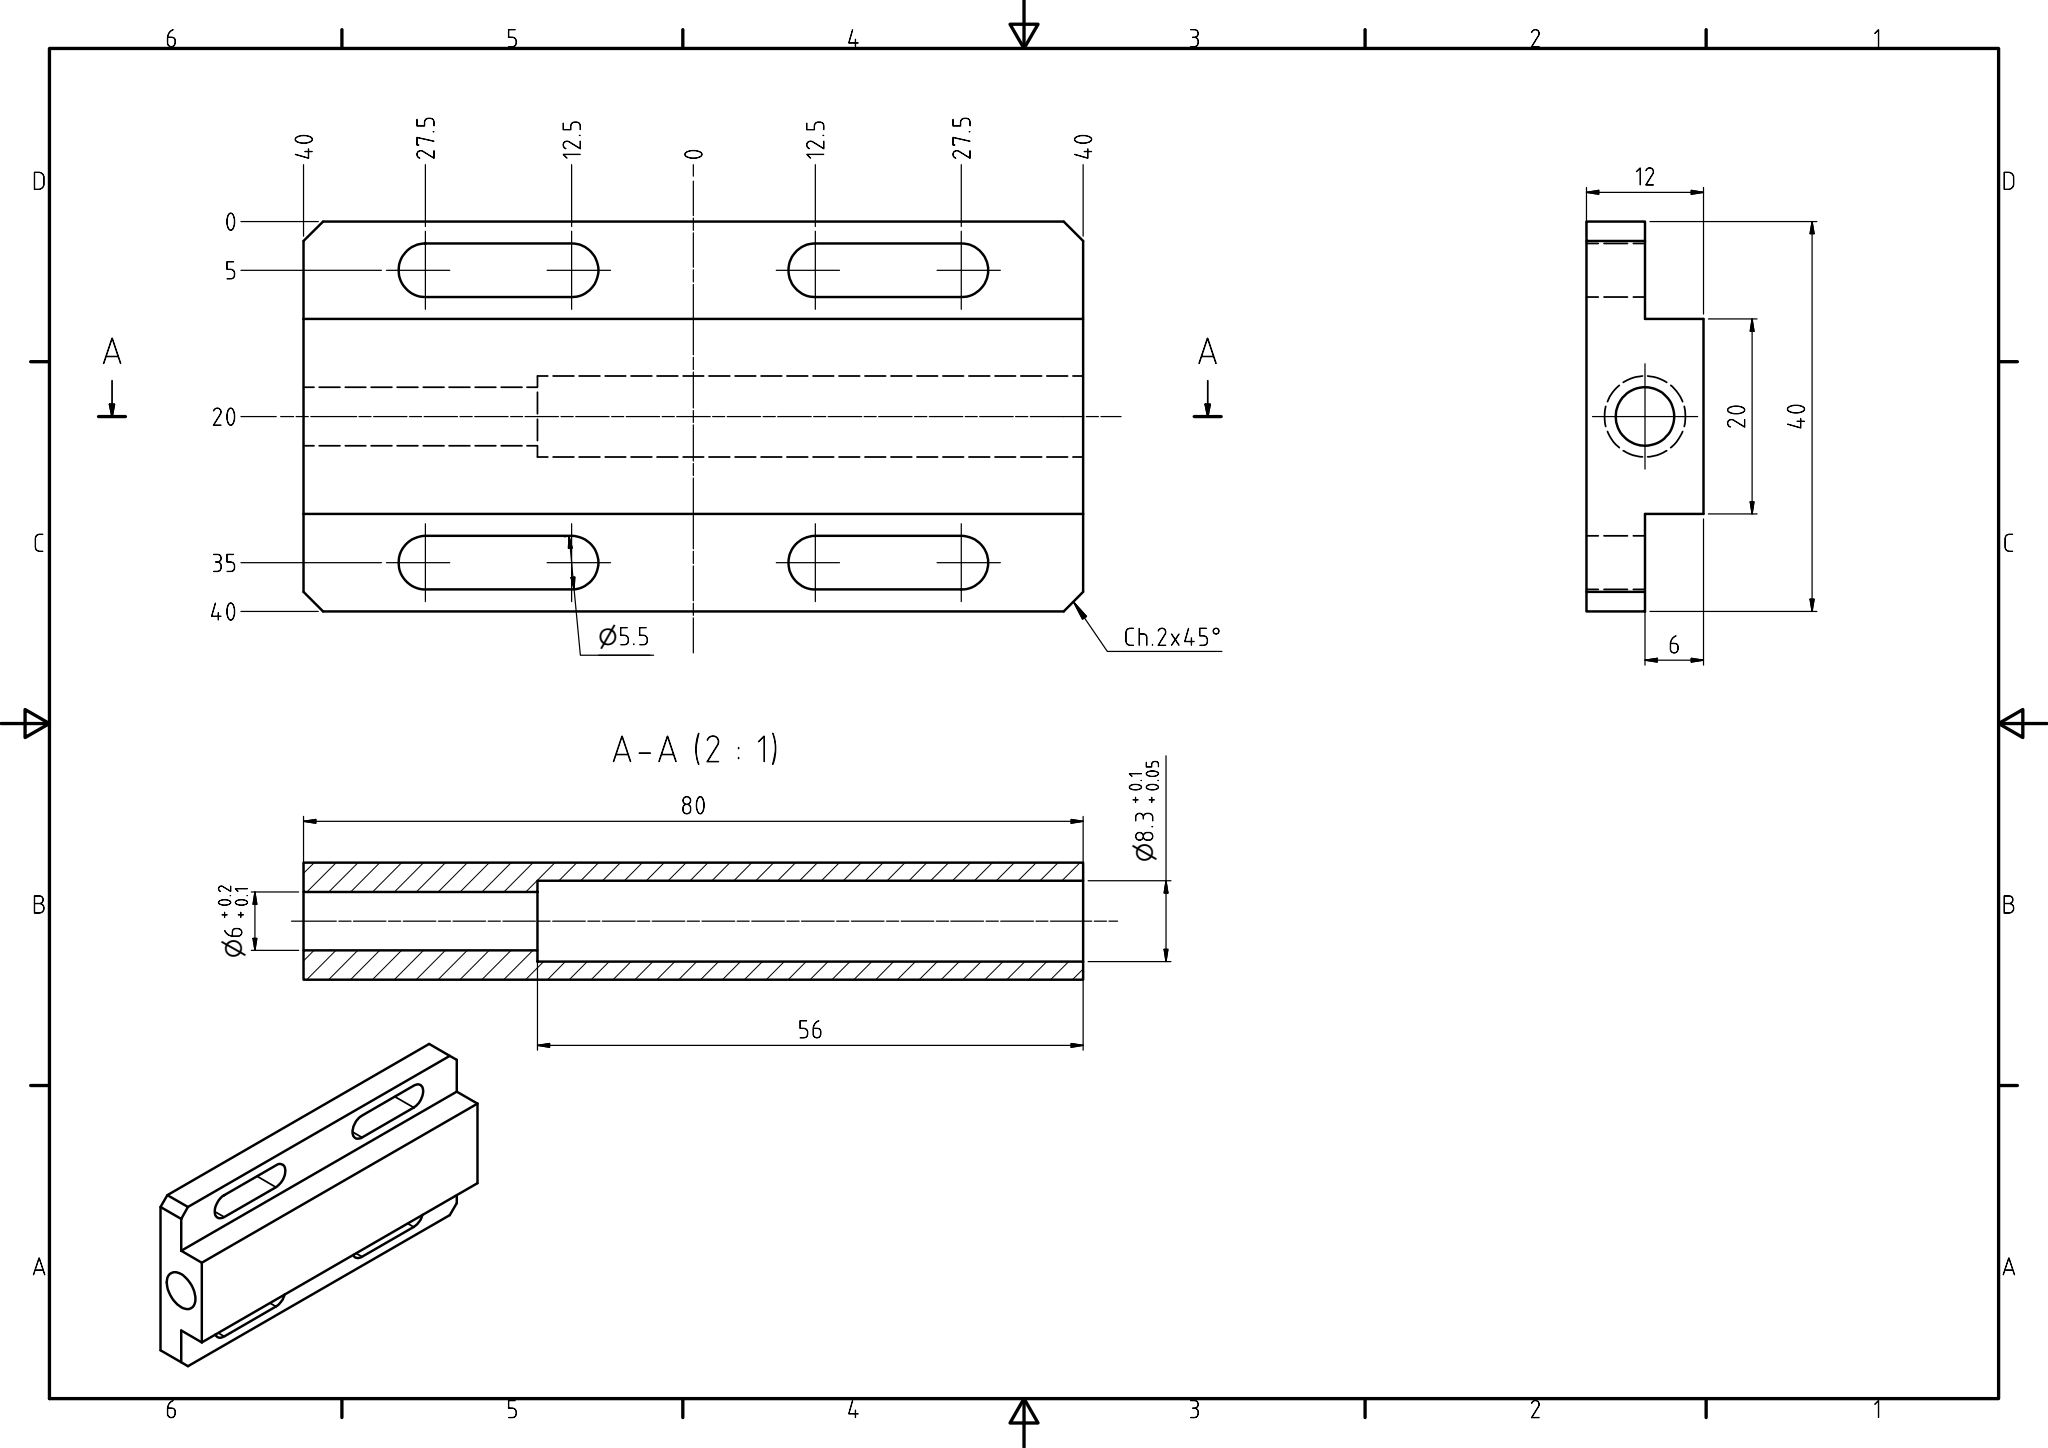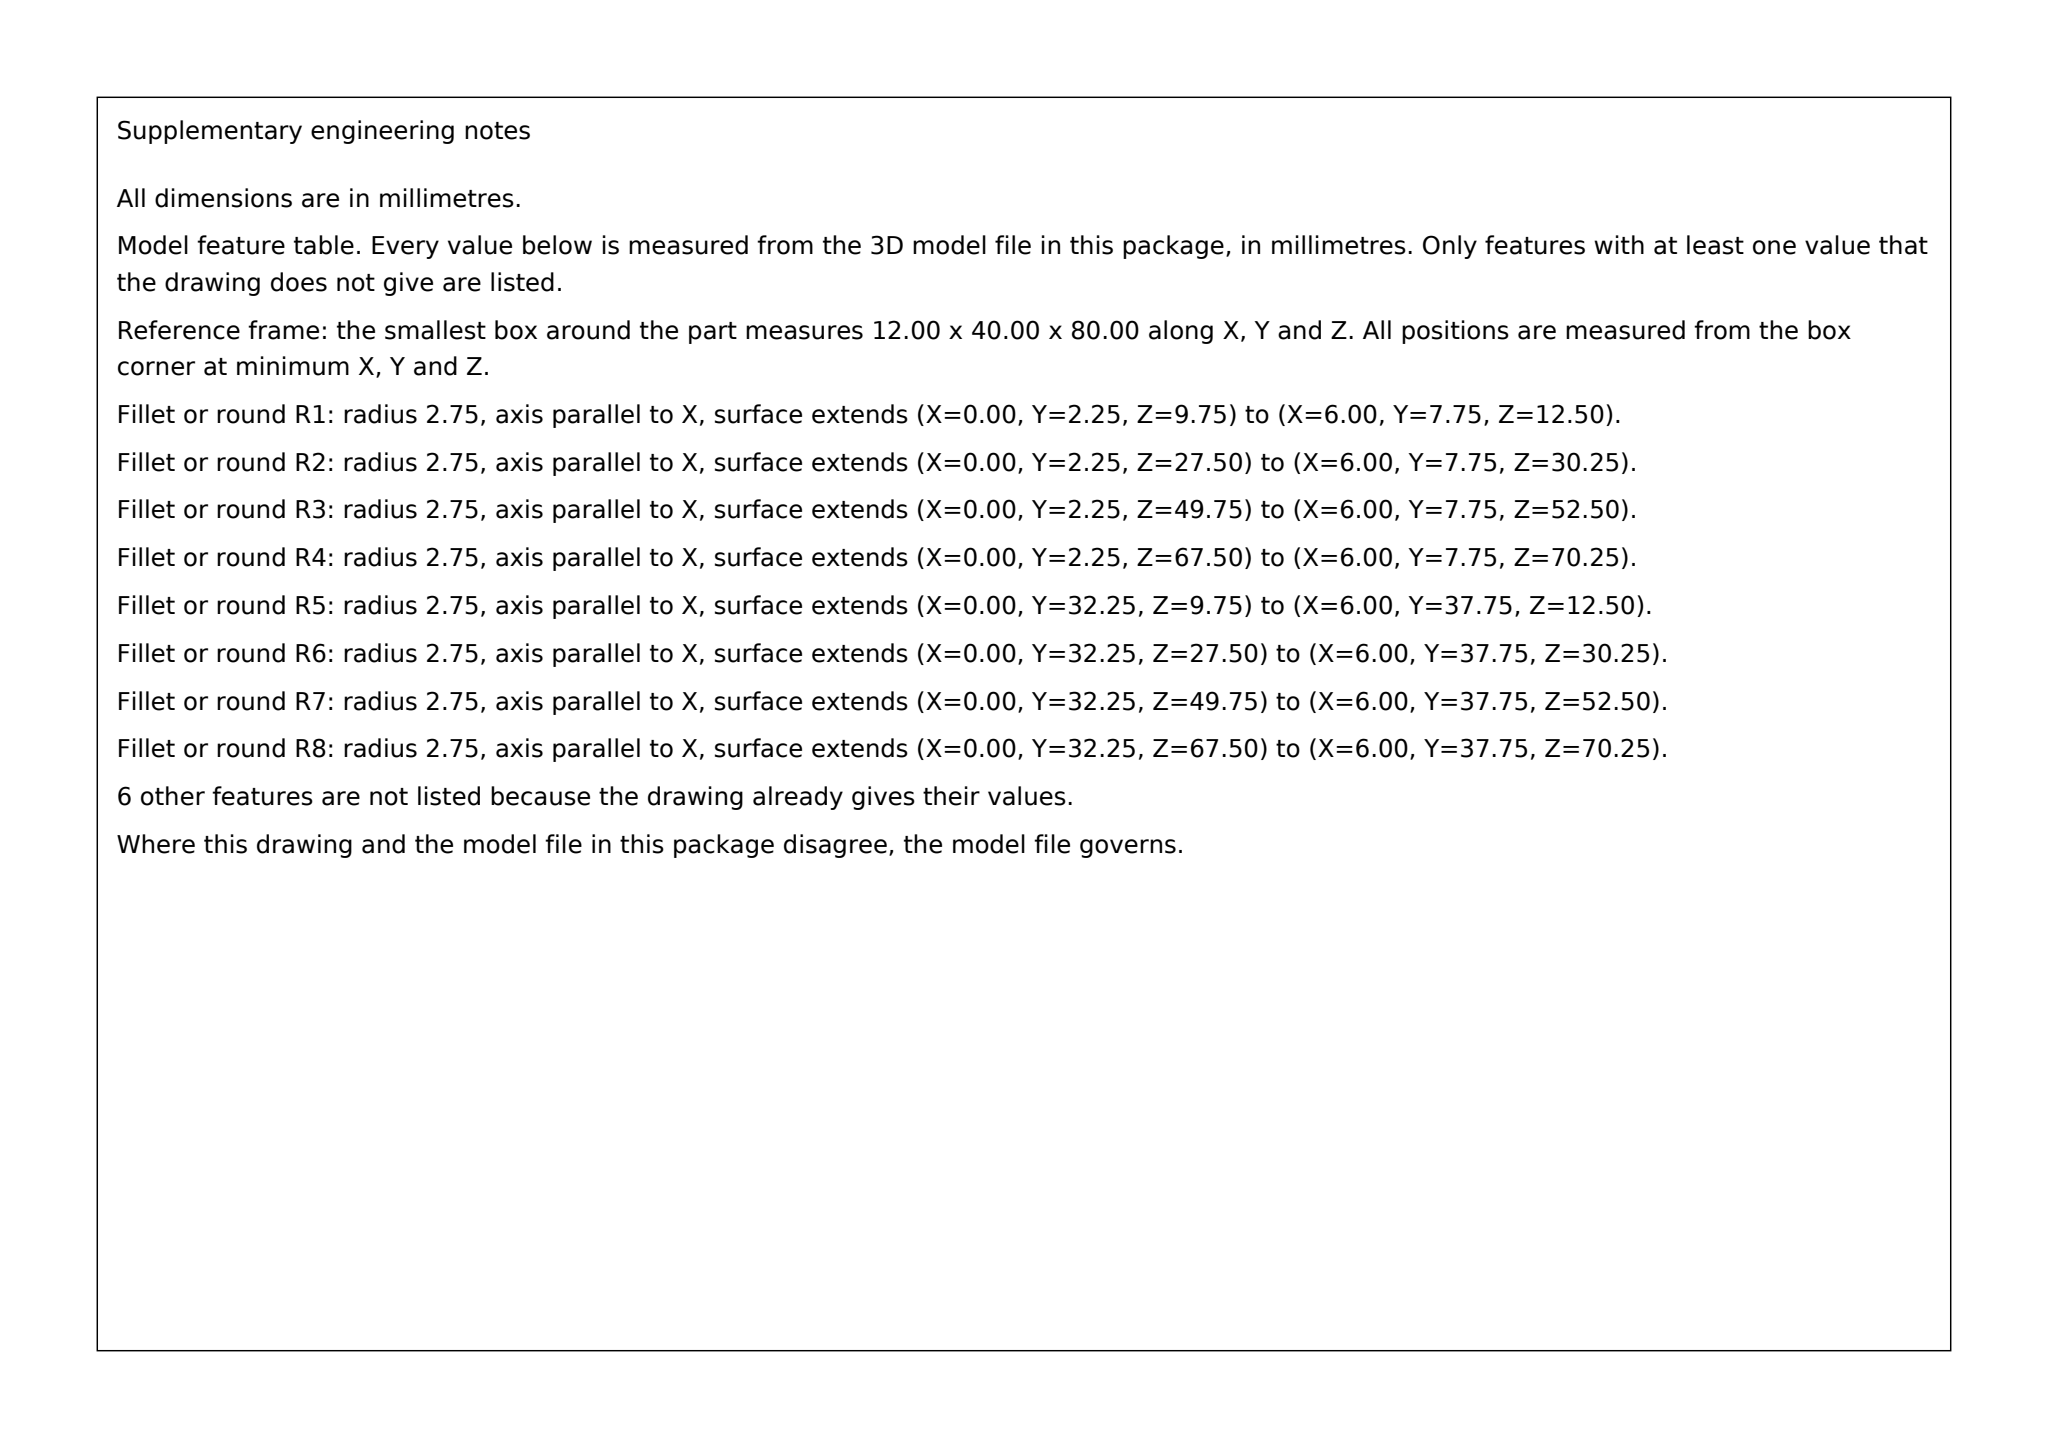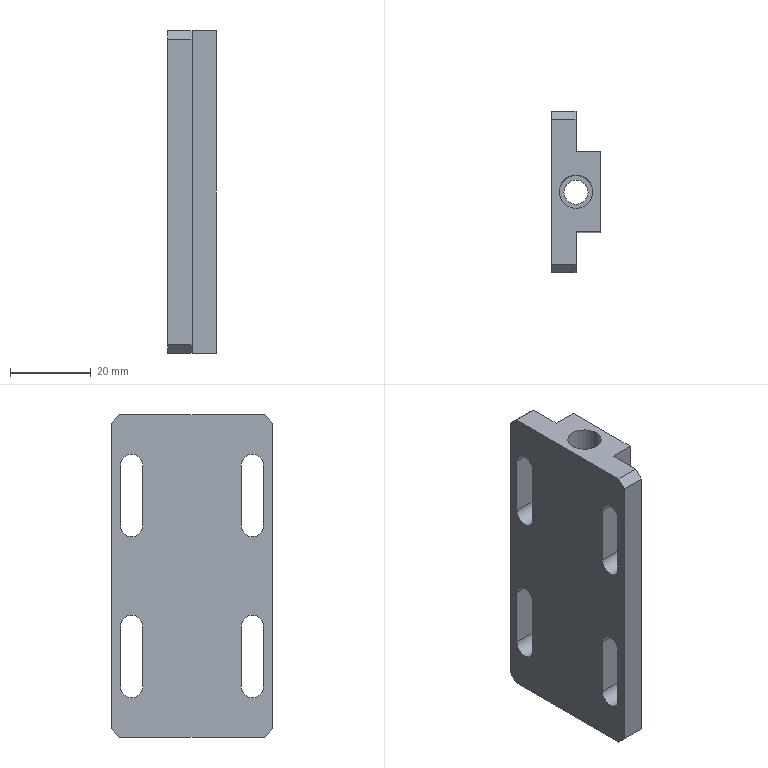Part | SolidWorks | mm | 1 solid | 35 faces | box 12 x 40 x 80 mm | volume 22493 mm3 | plane 23 | cylinder 12 | commonest cylinder face diameters 5.5 x8 6 x2 8.3 x2